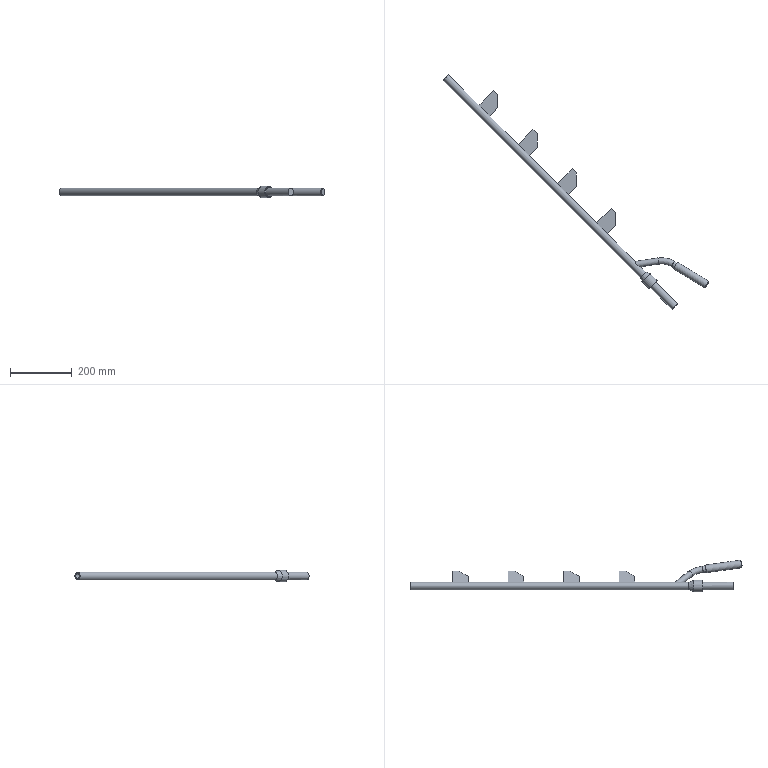Component | NX | POS_PUSH_ROD_2 | 1 solid | 42 faces | volume 485303 mm3 | plane 30 | cylinder 8 | cone 3 | torus 1 | commonest cylinder face diameters 25 x3 20 x2 17 x1 38 x1 30 x1